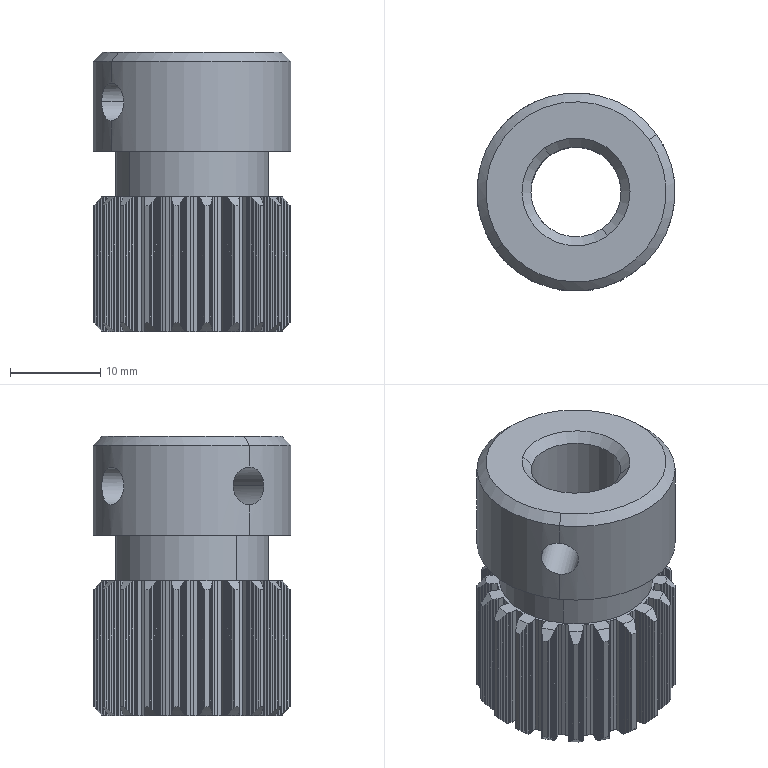Component | SolidWorks | Gear-1 | 1 solid | 580 faces | box 22 x 22 x 31 mm | volume 7158 mm3 | plane 504 | cone 46 | cylinder 30 | commonest cylinder face diameters 22 x22 4.2 x4 10 x2 17 x2
build123d program:
from build123d import *

# Parameters (mm, degrees)
F_4_2_4_2_DIAMETER_HOLE1_D     = 4.2
F_4_2_4_2_DIAMETER_HOLE1_DEPTH = 6.462
F_4_2_4_2_DIAMETER_HOLE2_D     = 4.2
F_4_2_4_2_DIAMETER_HOLE2_DEPTH = 6.462
GEAR_TEETH_M1_Z20_CUT_DEPTH    = 15.5


with BuildPart() as part:
    # Sketch1_2 → Revolve1 (revolve)
    with BuildSketch(Plane.XY):
        Polygon((-31, 10), (-31, 0), (0, 0), (0, 10), (-1, 11), (-11, 11), (-11, 8.5), (-16, 8.5), (-16, 10), (-17, 11), (-30, 11), align=None)
    revolve(axis=Axis((-31, 0, 0), (1, 0, 0)))

    # Sketch2 → Tapered Countersunk Hole 1 for M8 Flat H (revolve, cut)
    with BuildSketch(Plane(origin=(0, 0, 0), x_dir=(0, 0, -1), z_dir=(0, 1, 0))):
        Polygon((0, 0), (0, 31), (6, 31), (5, 30), (5, 1), (6, 0), align=None)
    revolve(axis=Axis((6.35, 0, 0), (-1, 0, 0)), mode=Mode.SUBTRACT)

    # 4.2 _4.2_ Diameter Hole1
    with Locations(Plane(origin=(0, 4.538, 0), x_dir=(-1, 0, 0), z_dir=(0, -1, 0))):
        with Locations((5.5, 0)):
            Hole(F_4_2_4_2_DIAMETER_HOLE1_D / 2, depth=F_4_2_4_2_DIAMETER_HOLE1_DEPTH)

    # 4.2 _4.2_ Diameter Hole2
    with Locations(Plane.XY.offset(-4.538)):
        with Locations((-5.5, 0)):
            Hole(F_4_2_4_2_DIAMETER_HOLE2_D / 2, depth=F_4_2_4_2_DIAMETER_HOLE2_DEPTH)

    # Sketch1 → Gear teeth m1 z20 cut (cut)
    with BuildSketch(Plane.ZY.offset(31)):
        Polygon((-1.417, 11.513), (-1.343, 10.918), (-1.23, 10.77), (-1.124, 10.62), (-1.025, 10.469), (-0.9324, 10.317), (-0.8477, 10.163), (-0.7711, 10.008), (-0.7033, 9.853), (-0.6451, 9.696), (-0.5985, 9.538), (-0.5689, 9.38), (-0.5298, 8.734), (-0.1297, 8.749), (0.2706, 8.746), (0.6704, 8.724), (0.7199, 9.369), (0.7521, 9.528), (0.8012, 9.684), (0.8618, 9.84), (0.9322, 9.995), (1.011, 10.148), (1.098, 10.3), (1.193, 10.451), (1.295, 10.601), (1.404, 10.748), (1.519, 10.895), (1.602, 11.489), align=None)
        Polygon((2.21, 11.387), (2.096, 10.798), (2.158, 10.623), (2.213, 10.448), (2.261, 10.273), (2.301, 10.1), (2.334, 9.928), (2.359, 9.757), (2.376, 9.588), (2.383, 9.421), (2.378, 9.257), (2.357, 9.096), (2.195, 8.47), (2.58, 8.361), (2.96, 8.234), (3.334, 8.09), (3.58, 8.688), (3.659, 8.829), (3.755, 8.963), (3.86, 9.092), (3.975, 9.218), (4.098, 9.339), (4.228, 9.457), (4.364, 9.571), (4.507, 9.682), (4.656, 9.789), (4.811, 9.892), (5.074, 10.431), align=None)
        Polygon((5.621, 10.147), (5.33, 9.622), (5.335, 9.436), (5.333, 9.252), (5.325, 9.072), (5.31, 8.894), (5.288, 8.72), (5.259, 8.55), (5.222, 8.384), (5.177, 8.224), (5.122, 8.069), (5.053, 7.923), (4.705, 7.377), (5.038, 7.154), (5.36, 6.916), (5.67, 6.664), (6.09, 7.157), (6.209, 7.266), (6.341, 7.364), (6.481, 7.454), (6.629, 7.538), (6.783, 7.616), (6.943, 7.688), (7.108, 7.754), (7.278, 7.815), (7.453, 7.871), (7.633, 7.921), (8.049, 8.353), align=None)
        Polygon((8.482, 7.913), (8.043, 7.504), (7.99, 7.326), (7.931, 7.152), (7.867, 6.982), (7.798, 6.818), (7.724, 6.66), (7.644, 6.507), (7.558, 6.36), (7.465, 6.221), (7.365, 6.091), (7.254, 5.974), (6.755, 5.562), (7.002, 5.248), (7.235, 4.922), (7.452, 4.586), (8.003, 4.925), (8.15, 4.992), (8.306, 5.044), (8.467, 5.087), (8.634, 5.121), (8.804, 5.147), (8.979, 5.166), (9.156, 5.178), (9.337, 5.183), (9.521, 5.182), (9.707, 5.175), (10.236, 5.457), align=None)
        Polygon((10.512, 4.905), (9.968, 4.651), (9.862, 4.498), (9.753, 4.351), (9.64, 4.21), (9.524, 4.075), (9.404, 3.947), (9.28, 3.826), (9.153, 3.714), (9.022, 3.61), (8.887, 3.517), (8.745, 3.44), (8.143, 3.203), (8.281, 2.827), (8.401, 2.445), (8.504, 2.058), (9.133, 2.211), (9.294, 2.229), (9.458, 2.231), (9.625, 2.221), (9.794, 2.202), (9.964, 2.174), (10.136, 2.138), (10.308, 2.095), (10.482, 2.044), (10.656, 1.986), (10.831, 1.922), (11.422, 2.027), align=None)
        Polygon((11.513, 1.417), (10.918, 1.343), (10.77, 1.23), (10.62, 1.124), (10.469, 1.025), (10.317, 0.9324), (10.163, 0.8477), (10.008, 0.7711), (9.853, 0.7033), (9.696, 0.6451), (9.538, 0.5985), (9.38, 0.5689), (8.734, 0.5298), (8.749, 0.1297), (8.746, -0.2706), (8.724, -0.6704), (9.369, -0.7199), (9.528, -0.7521), (9.684, -0.8012), (9.84, -0.8618), (9.995, -0.9322), (10.148, -1.011), (10.3, -1.098), (10.451, -1.193), (10.601, -1.295), (10.748, -1.404), (10.895, -1.519), (11.489, -1.602), align=None)
        Polygon((11.387, -2.21), (10.798, -2.096), (10.623, -2.158), (10.448, -2.213), (10.273, -2.261), (10.1, -2.301), (9.928, -2.334), (9.757, -2.359), (9.588, -2.376), (9.421, -2.383), (9.257, -2.378), (9.096, -2.357), (8.47, -2.195), (8.361, -2.58), (8.234, -2.96), (8.09, -3.334), (8.688, -3.58), (8.829, -3.659), (8.963, -3.755), (9.092, -3.86), (9.218, -3.975), (9.339, -4.098), (9.457, -4.228), (9.571, -4.364), (9.682, -4.507), (9.789, -4.656), (9.892, -4.811), (10.431, -5.074), align=None)
        Polygon((10.147, -5.621), (9.622, -5.33), (9.436, -5.335), (9.252, -5.333), (9.072, -5.325), (8.894, -5.31), (8.72, -5.288), (8.55, -5.259), (8.384, -5.222), (8.224, -5.177), (8.069, -5.122), (7.923, -5.053), (7.377, -4.705), (7.154, -5.038), (6.916, -5.36), (6.664, -5.67), (7.157, -6.09), (7.266, -6.209), (7.364, -6.341), (7.454, -6.481), (7.538, -6.629), (7.616, -6.783), (7.688, -6.943), (7.754, -7.108), (7.815, -7.278), (7.871, -7.453), (7.921, -7.633), (8.353, -8.049), align=None)
        Polygon((7.913, -8.482), (7.504, -8.043), (7.326, -7.99), (7.152, -7.931), (6.982, -7.867), (6.818, -7.798), (6.66, -7.724), (6.507, -7.644), (6.36, -7.558), (6.221, -7.465), (6.091, -7.365), (5.974, -7.254), (5.562, -6.755), (5.248, -7.002), (4.922, -7.235), (4.586, -7.452), (4.925, -8.003), (4.992, -8.15), (5.044, -8.306), (5.087, -8.467), (5.121, -8.634), (5.147, -8.804), (5.166, -8.979), (5.178, -9.156), (5.183, -9.337), (5.182, -9.521), (5.175, -9.707), (5.457, -10.236), align=None)
        Polygon((4.905, -10.512), (4.651, -9.968), (4.498, -9.862), (4.351, -9.753), (4.21, -9.64), (4.075, -9.524), (3.947, -9.404), (3.826, -9.28), (3.714, -9.153), (3.61, -9.022), (3.517, -8.887), (3.44, -8.745), (3.203, -8.143), (2.827, -8.281), (2.445, -8.401), (2.058, -8.504), (2.211, -9.133), (2.229, -9.294), (2.231, -9.458), (2.221, -9.625), (2.202, -9.794), (2.174, -9.964), (2.138, -10.136), (2.095, -10.308), (2.044, -10.482), (1.986, -10.656), (1.922, -10.831), (2.027, -11.422), align=None)
        Polygon((1.417, -11.513), (1.343, -10.918), (1.23, -10.77), (1.124, -10.62), (1.025, -10.469), (0.9324, -10.317), (0.8477, -10.163), (0.7711, -10.008), (0.7033, -9.853), (0.6451, -9.696), (0.5985, -9.538), (0.5689, -9.38), (0.5298, -8.734), (0.1297, -8.749), (-0.2706, -8.746), (-0.6704, -8.724), (-0.7199, -9.369), (-0.7521, -9.528), (-0.8012, -9.684), (-0.8618, -9.84), (-0.9322, -9.995), (-1.011, -10.148), (-1.098, -10.3), (-1.193, -10.451), (-1.295, -10.601), (-1.404, -10.748), (-1.519, -10.895), (-1.602, -11.489), align=None)
        Polygon((-2.21, -11.387), (-2.096, -10.798), (-2.158, -10.623), (-2.213, -10.448), (-2.261, -10.273), (-2.301, -10.1), (-2.334, -9.928), (-2.359, -9.757), (-2.376, -9.588), (-2.383, -9.421), (-2.378, -9.257), (-2.357, -9.096), (-2.195, -8.47), (-2.58, -8.361), (-2.96, -8.234), (-3.334, -8.09), (-3.58, -8.688), (-3.659, -8.829), (-3.755, -8.963), (-3.86, -9.092), (-3.975, -9.218), (-4.098, -9.339), (-4.228, -9.457), (-4.364, -9.571), (-4.507, -9.682), (-4.656, -9.789), (-4.811, -9.892), (-5.074, -10.431), align=None)
        Polygon((-5.621, -10.147), (-5.33, -9.622), (-5.335, -9.436), (-5.333, -9.252), (-5.325, -9.072), (-5.31, -8.894), (-5.288, -8.72), (-5.259, -8.55), (-5.222, -8.384), (-5.177, -8.224), (-5.122, -8.069), (-5.053, -7.923), (-4.705, -7.377), (-5.038, -7.154), (-5.36, -6.916), (-5.67, -6.664), (-6.09, -7.157), (-6.209, -7.266), (-6.341, -7.364), (-6.481, -7.454), (-6.629, -7.538), (-6.783, -7.616), (-6.943, -7.688), (-7.108, -7.754), (-7.278, -7.815), (-7.453, -7.871), (-7.633, -7.921), (-8.049, -8.353), align=None)
        Polygon((-8.482, -7.913), (-8.043, -7.504), (-7.99, -7.326), (-7.931, -7.152), (-7.867, -6.982), (-7.798, -6.818), (-7.724, -6.66), (-7.644, -6.507), (-7.558, -6.36), (-7.465, -6.221), (-7.365, -6.091), (-7.254, -5.974), (-6.755, -5.562), (-7.002, -5.248), (-7.235, -4.922), (-7.452, -4.586), (-8.003, -4.925), (-8.15, -4.992), (-8.306, -5.044), (-8.467, -5.087), (-8.634, -5.121), (-8.804, -5.147), (-8.979, -5.166), (-9.156, -5.178), (-9.337, -5.183), (-9.521, -5.182), (-9.707, -5.175), (-10.236, -5.457), align=None)
        Polygon((-10.512, -4.905), (-9.968, -4.651), (-9.862, -4.498), (-9.753, -4.351), (-9.64, -4.21), (-9.524, -4.075), (-9.404, -3.947), (-9.28, -3.826), (-9.153, -3.714), (-9.022, -3.61), (-8.887, -3.517), (-8.745, -3.44), (-8.143, -3.203), (-8.281, -2.827), (-8.401, -2.445), (-8.504, -2.058), (-9.133, -2.211), (-9.294, -2.229), (-9.458, -2.231), (-9.625, -2.221), (-9.794, -2.202), (-9.964, -2.174), (-10.136, -2.138), (-10.308, -2.095), (-10.482, -2.044), (-10.656, -1.986), (-10.831, -1.922), (-11.422, -2.027), align=None)
        Polygon((-11.513, -1.417), (-10.918, -1.343), (-10.77, -1.23), (-10.62, -1.124), (-10.469, -1.025), (-10.317, -0.9324), (-10.163, -0.8477), (-10.008, -0.7711), (-9.853, -0.7033), (-9.696, -0.6451), (-9.538, -0.5985), (-9.38, -0.5689), (-8.734, -0.5298), (-8.749, -0.1297), (-8.746, 0.2706), (-8.724, 0.6704), (-9.369, 0.7199), (-9.528, 0.7521), (-9.684, 0.8012), (-9.84, 0.8618), (-9.995, 0.9322), (-10.148, 1.011), (-10.3, 1.098), (-10.451, 1.193), (-10.601, 1.295), (-10.748, 1.404), (-10.895, 1.519), (-11.489, 1.602), align=None)
        Polygon((-11.387, 2.21), (-10.798, 2.096), (-10.623, 2.158), (-10.448, 2.213), (-10.273, 2.261), (-10.1, 2.301), (-9.928, 2.334), (-9.757, 2.359), (-9.588, 2.376), (-9.421, 2.383), (-9.257, 2.378), (-9.096, 2.357), (-8.47, 2.195), (-8.361, 2.58), (-8.234, 2.96), (-8.09, 3.334), (-8.688, 3.58), (-8.829, 3.659), (-8.963, 3.755), (-9.092, 3.86), (-9.218, 3.975), (-9.339, 4.098), (-9.457, 4.228), (-9.571, 4.364), (-9.682, 4.507), (-9.789, 4.656), (-9.892, 4.811), (-10.431, 5.074), align=None)
        Polygon((-10.147, 5.621), (-9.622, 5.33), (-9.436, 5.335), (-9.252, 5.333), (-9.072, 5.325), (-8.894, 5.31), (-8.72, 5.288), (-8.55, 5.259), (-8.384, 5.222), (-8.224, 5.177), (-8.069, 5.122), (-7.923, 5.053), (-7.377, 4.705), (-7.154, 5.038), (-6.916, 5.36), (-6.664, 5.67), (-7.157, 6.09), (-7.266, 6.209), (-7.364, 6.341), (-7.454, 6.481), (-7.538, 6.629), (-7.616, 6.783), (-7.688, 6.943), (-7.754, 7.108), (-7.815, 7.278), (-7.871, 7.453), (-7.921, 7.633), (-8.353, 8.049), align=None)
        Polygon((-7.913, 8.482), (-7.504, 8.043), (-7.326, 7.99), (-7.152, 7.931), (-6.982, 7.867), (-6.818, 7.798), (-6.66, 7.724), (-6.507, 7.644), (-6.36, 7.558), (-6.221, 7.465), (-6.091, 7.365), (-5.974, 7.254), (-5.562, 6.755), (-5.248, 7.002), (-4.922, 7.235), (-4.586, 7.452), (-4.925, 8.003), (-4.992, 8.15), (-5.044, 8.306), (-5.087, 8.467), (-5.121, 8.634), (-5.147, 8.804), (-5.166, 8.979), (-5.178, 9.156), (-5.183, 9.337), (-5.182, 9.521), (-5.175, 9.707), (-5.457, 10.236), align=None)
        Polygon((-4.905, 10.512), (-4.651, 9.968), (-4.498, 9.862), (-4.351, 9.753), (-4.21, 9.64), (-4.075, 9.524), (-3.947, 9.404), (-3.826, 9.28), (-3.714, 9.153), (-3.61, 9.022), (-3.517, 8.887), (-3.44, 8.745), (-3.203, 8.143), (-2.827, 8.281), (-2.445, 8.401), (-2.058, 8.504), (-2.211, 9.133), (-2.229, 9.294), (-2.231, 9.458), (-2.221, 9.625), (-2.202, 9.794), (-2.174, 9.964), (-2.138, 10.136), (-2.095, 10.308), (-2.044, 10.482), (-1.986, 10.656), (-1.922, 10.831), (-2.027, 11.422), align=None)
    extrude(amount=-GEAR_TEETH_M1_Z20_CUT_DEPTH, mode=Mode.SUBTRACT)


solid = part.part

# Placed as in the assembly
solid = solid.moved(Location((-180.767, 560.9, -231.5), (90, 35.46, 90)))